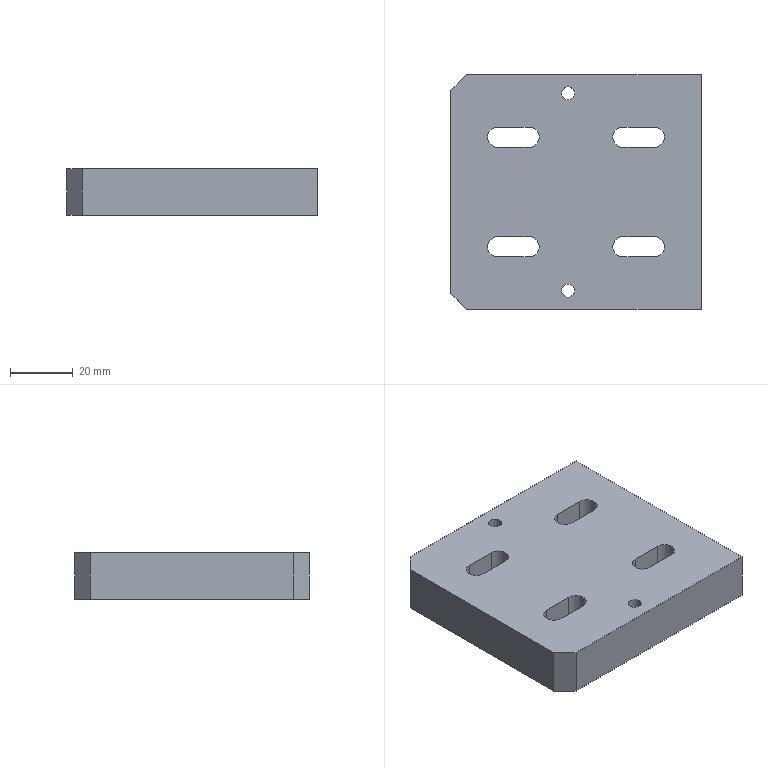CAM job | Mastercam | mm | 10 operations | part box 80 x 75 x 15
1. Facing | 20 - 63 平铣刀
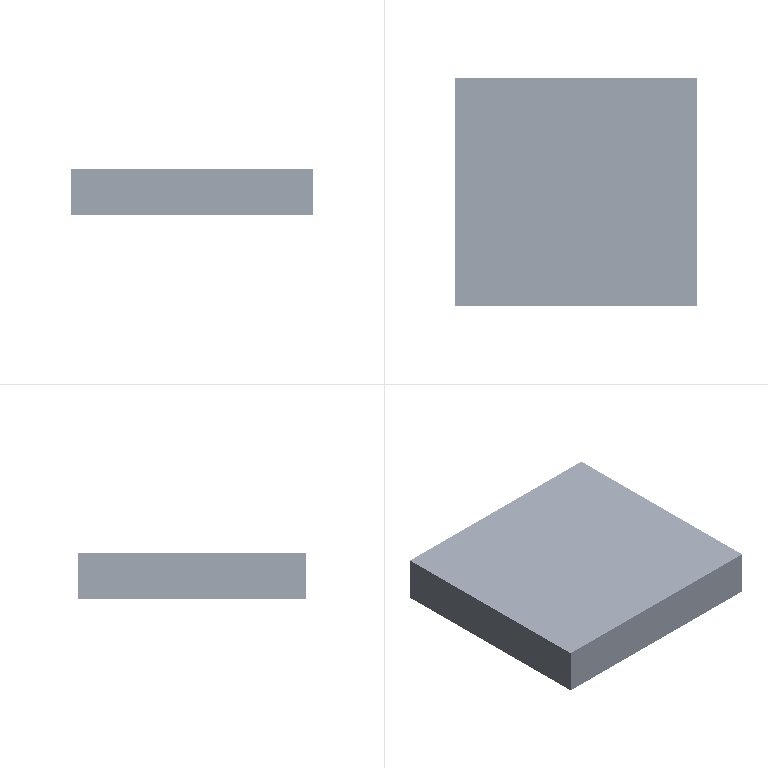2. Contour (Ramp) | 9 - 10 平铣刀
3. Contour (2D) | 10 - 10 平铣刀
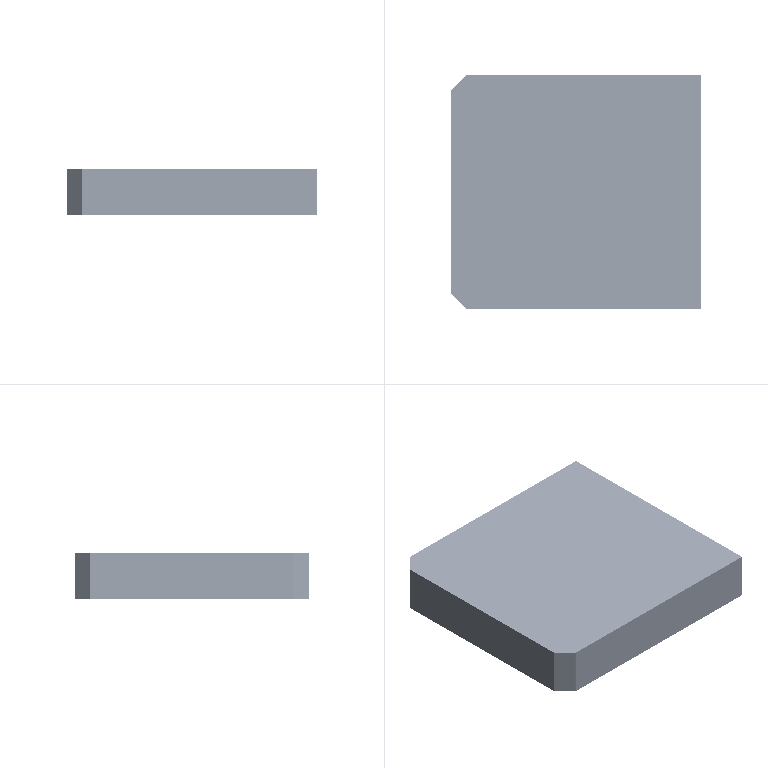4. Contour (Ramp) | 4 - 4 平铣刀
5. Contour (Ramp) | 4 - 4 平铣刀
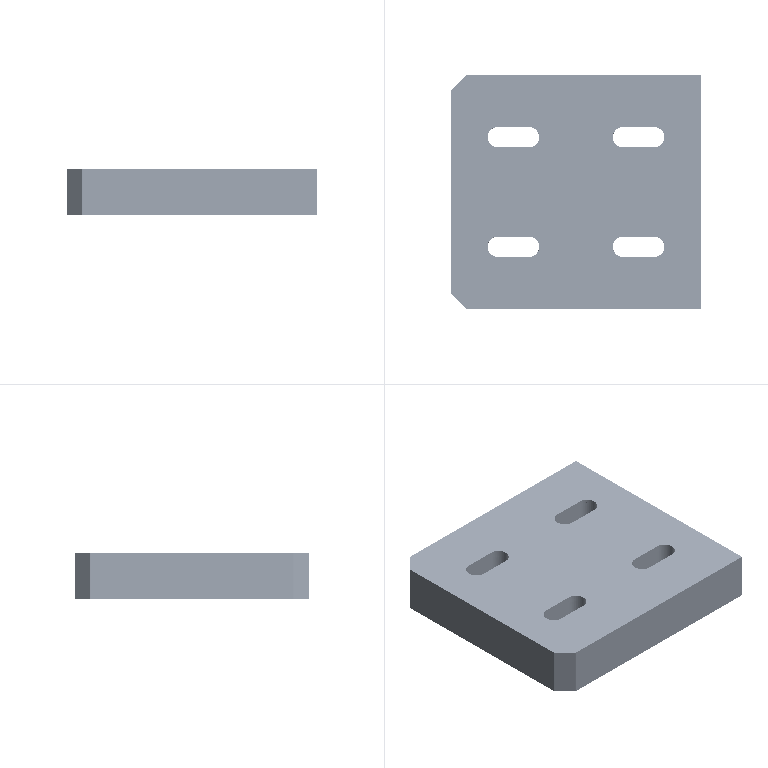6. Drill/Counterbore | 7 - 4 倒角刀
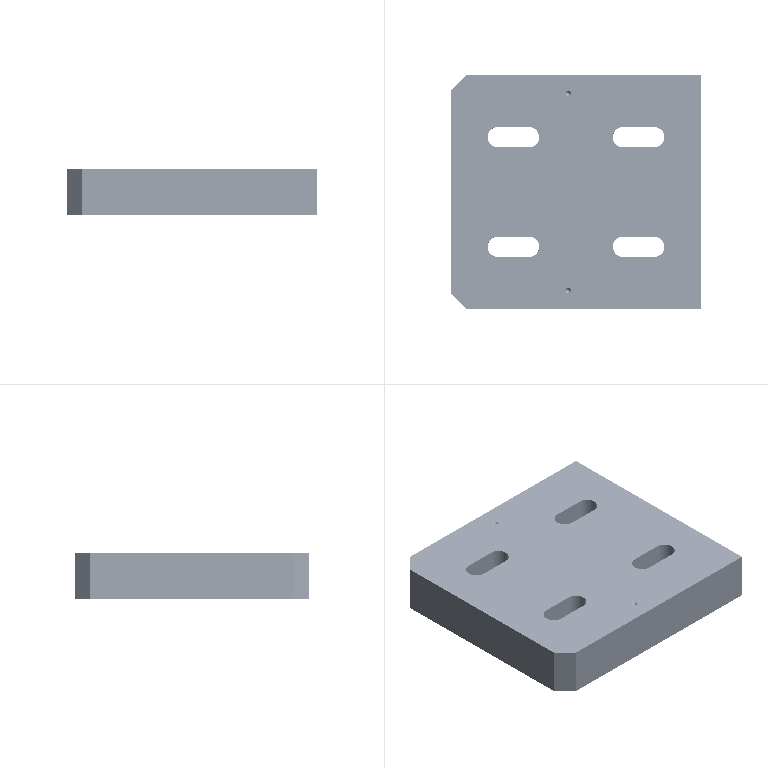7. Contour (2D chamfer) | 7 - 4 倒角刀
8. Facing | 20 - 63 平铣刀
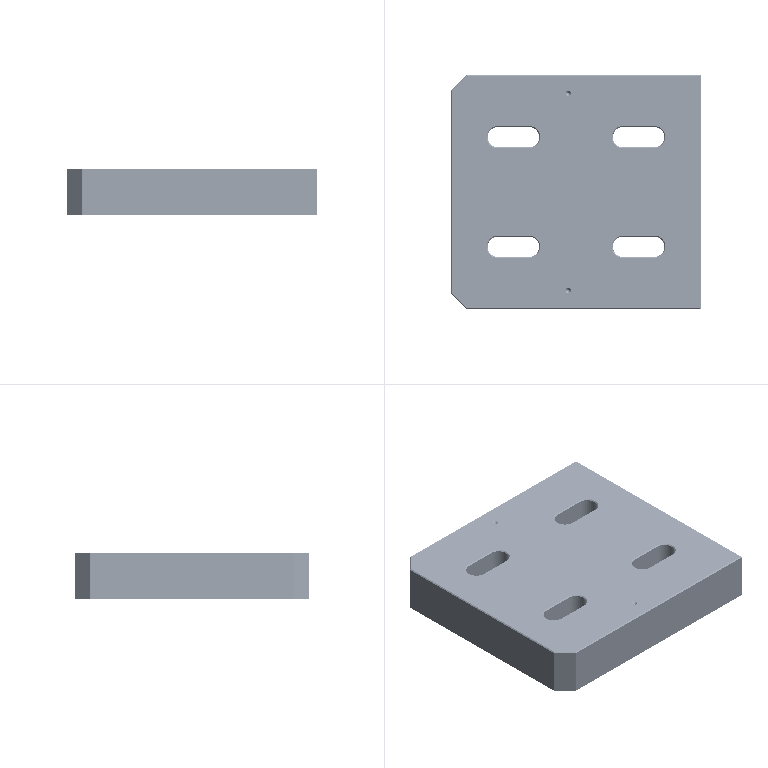9. Contour (2D chamfer) | 7 - 4 倒角刀
10. Drill/Counterbore | 7 - 4 倒角刀